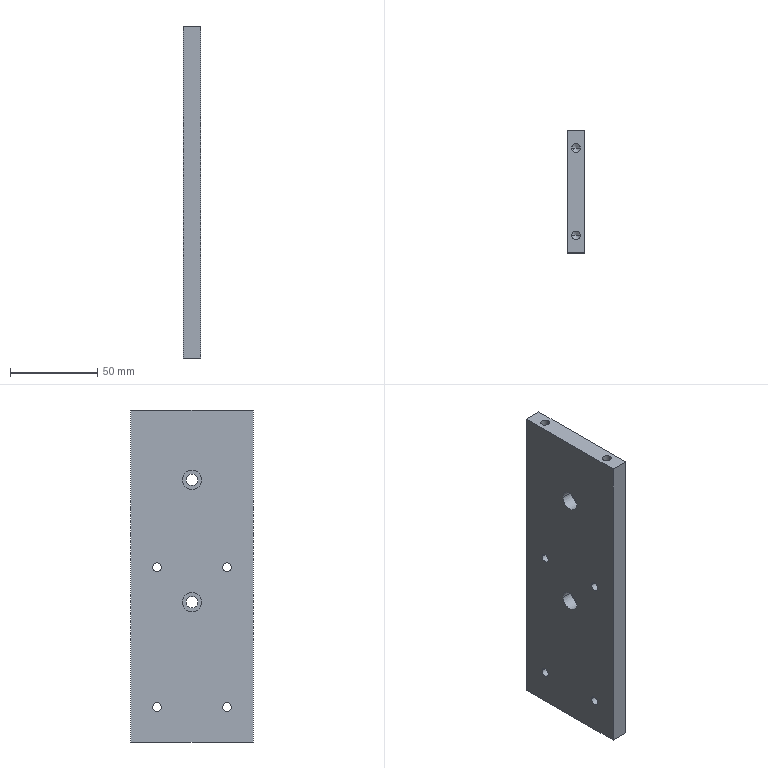Component | SolidWorks | 01-05MarkingMachineMountingVerticalPlate-1 | 1 solid | 32 faces | box 10 x 70 x 190 mm | volume 130094 mm3 | cylinder 20 | plane 8 | cone 4 | commonest cylinder face diameters 5 x12 11 x4 6.6 x4 | material A3 Steel
build123d program:
from build123d import *

# Parameters (mm, degrees)
SKETCH1_W                                          = 70
SKETCH1_H                                          = 190
BOSS_EXTRUDE1_DEPTH                                = 5
M6_TAPPED_HOLE1_D                                  = 5
M6_TAPPED_HOLE1_DEPTH                              = 15
M6_TAPPED_HOLE1_TIP                                = 1.502
HOLE_SIZE_ACCORDING_TO_TYPE_1_OF_HEXAG_D           = 6.6
HOLE_SIZE_ACCORDING_TO_TYPE_1_OF_HEXAG_CBORE_D     = 11
HOLE_SIZE_ACCORDING_TO_TYPE_1_OF_HEXAG_CBORE_DEPTH = 6.8
M6_TAPPED_HOLE2_D                                  = 5


with BuildPart() as part:
    # Sketch1 → Boss-Extrude1 (new, symmetric)
    with BuildSketch(Plane.XY):
        Rectangle(SKETCH1_W, SKETCH1_H)
    extrude(amount=BOSS_EXTRUDE1_DEPTH, both=True)

    # M6 Tapped Hole1
    with Locations(Plane(origin=(-25, -95, 0), x_dir=(0, 0, -1), z_dir=(0, -1, 0))):
        with Locations((0, 0), (0, 50)):
            Hole(M6_TAPPED_HOLE1_D / 2, depth=M6_TAPPED_HOLE1_DEPTH)
            with Locations((0, 0, -(M6_TAPPED_HOLE1_DEPTH + M6_TAPPED_HOLE1_TIP / 2))):  # 118° drill point
                Cone(0, M6_TAPPED_HOLE1_D / 2, M6_TAPPED_HOLE1_TIP, mode=Mode.SUBTRACT)

    # Hole Size _According to_ Type 1 of Hexag (through all)
    with Locations(Plane(origin=(0, 15, 5), x_dir=(1, 0, 0), z_dir=(0, 0, 1))):
        with Locations((0, 0), (0, -70)):
            CounterBoreHole(HOLE_SIZE_ACCORDING_TO_TYPE_1_OF_HEXAG_D / 2, HOLE_SIZE_ACCORDING_TO_TYPE_1_OF_HEXAG_CBORE_D / 2, HOLE_SIZE_ACCORDING_TO_TYPE_1_OF_HEXAG_CBORE_DEPTH)

    # M6 Tapped Hole2 (through all)
    with Locations(Plane(origin=(-20, -5, 5), x_dir=(1, 0, 0), z_dir=(0, 0, 1))):
        with Locations((0, 0), (0, 80), (40, 80), (40, 0)):
            Hole(M6_TAPPED_HOLE2_D / 2)


solid = part.part

# Placed as in the assembly
solid = solid.moved(Location((-51.91, 2.41, -10), (-90, -90, 0)))
STEP:
#1=CARTESIAN_POINT('',(-1.847,-0.7909,-0.1969));
#2=VERTEX_POINT('',#1);
#3=CARTESIAN_POINT('',(-1.847,-0.5941,-0.1969));
#4=VERTEX_POINT('',#3);
#5=CARTESIAN_POINT('',(-1.847,-0.6925,-0.1969));
#6=DIRECTION('',(-1.,0.,0.));
#7=DIRECTION('',(0.,1.,0.));
#8=AXIS2_PLACEMENT_3D('',#5,#6,#7);
#9=CIRCLE('',#8,0.09843);
#10=EDGE_CURVE('',#2,#4,#9,.T.);
#11=ORIENTED_EDGE('',*,*,#10,.F.);
#12=CARTESIAN_POINT('',(-2.241,-0.7909,-0.1969));
#13=VERTEX_POINT('',#12);
#14=CARTESIAN_POINT('',(-2.241,-0.7909,-0.1969));
#15=DIRECTION('',(-1.,0.,0.));
#16=VECTOR('',#15,39.37);
#17=LINE('',#14,#16);
#18=EDGE_CURVE('',#2,#13,#17,.T.);
#19=ORIENTED_EDGE('',*,*,#18,.T.);
#20=CARTESIAN_POINT('',(-2.241,-0.5941,-0.1969));
#21=VERTEX_POINT('',#20);
#22=CARTESIAN_POINT('',(-2.241,-0.6925,-0.1969));
#23=DIRECTION('',(-1.,0.,0.));
#24=DIRECTION('',(0.,1.,0.));
#25=AXIS2_PLACEMENT_3D('',#22,#23,#24);
#26=CIRCLE('',#25,0.09843);
#27=EDGE_CURVE('',#13,#21,#26,.T.);
#28=ORIENTED_EDGE('',*,*,#27,.T.);
#29=CARTESIAN_POINT('',(-2.241,-0.5941,-0.1969));
#30=DIRECTION('',(-1.,0.,0.));
#31=VECTOR('',#30,39.37);
#32=LINE('',#29,#31);
#33=EDGE_CURVE('',#4,#21,#32,.T.);
#34=ORIENTED_EDGE('',*,*,#33,.F.);
#35=EDGE_LOOP('',(#11,#19,#28,#34));
#36=FACE_OUTER_BOUND('',#35,.T.);
#37=CARTESIAN_POINT('',(-2.241,-0.6925,-0.1969));
#38=DIRECTION('',(-1.,0.,0.));
#39=DIRECTION('',(0.,1.,0.));
#40=AXIS2_PLACEMENT_3D('',#37,#38,#39);
#41=CYLINDRICAL_SURFACE('',#40,0.09843);
#42=ADVANCED_FACE('',(#36),#41,.F.);
#43=CARTESIAN_POINT('',(-1.847,-0.7909,-3.346));
#44=VERTEX_POINT('',#43);
#45=CARTESIAN_POINT('',(-1.847,-0.5941,-3.346));
#46=VERTEX_POINT('',#45);
#47=CARTESIAN_POINT('',(-1.847,-0.6925,-3.346));
#48=DIRECTION('',(-1.,0.,0.));
#49=DIRECTION('',(0.,1.,0.));
#50=AXIS2_PLACEMENT_3D('',#47,#48,#49);
#51=CIRCLE('',#50,0.09843);
#52=EDGE_CURVE('',#44,#46,#51,.T.);
#53=ORIENTED_EDGE('',*,*,#52,.F.);
#54=CARTESIAN_POINT('',(-2.241,-0.7909,-3.346));
#55=VERTEX_POINT('',#54);
#56=CARTESIAN_POINT('',(-2.241,-0.7909,-3.346));
#57=DIRECTION('',(-1.,0.,0.));
#58=VECTOR('',#57,39.37);
#59=LINE('',#56,#58);
#60=EDGE_CURVE('',#44,#55,#59,.T.);
#61=ORIENTED_EDGE('',*,*,#60,.T.);
#62=CARTESIAN_POINT('',(-2.241,-0.5941,-3.346));
#63=VERTEX_POINT('',#62);
#64=CARTESIAN_POINT('',(-2.241,-0.6925,-3.346));
#65=DIRECTION('',(-1.,0.,0.));
#66=DIRECTION('',(0.,1.,0.));
#67=AXIS2_PLACEMENT_3D('',#64,#65,#66);
#68=CIRCLE('',#67,0.09843);
#69=EDGE_CURVE('',#55,#63,#68,.T.);
#70=ORIENTED_EDGE('',*,*,#69,.T.);
#71=CARTESIAN_POINT('',(-2.241,-0.5941,-3.346));
#72=DIRECTION('',(-1.,0.,0.));
#73=VECTOR('',#72,39.37);
#74=LINE('',#71,#73);
#75=EDGE_CURVE('',#46,#63,#74,.T.);
#76=ORIENTED_EDGE('',*,*,#75,.F.);
#77=EDGE_LOOP('',(#53,#61,#70,#76));
#78=FACE_OUTER_BOUND('',#77,.T.);
#79=CARTESIAN_POINT('',(-2.241,-0.6925,-3.346));
#80=DIRECTION('',(-1.,0.,0.));
#81=DIRECTION('',(0.,1.,0.));
#82=AXIS2_PLACEMENT_3D('',#79,#80,#81);
#83=CYLINDRICAL_SURFACE('',#82,0.09843);
#84=ADVANCED_FACE('',(#78),#83,.F.);
#85=CARTESIAN_POINT('',(-1.847,0.7839,-3.346));
#86=VERTEX_POINT('',#85);
#87=CARTESIAN_POINT('',(-1.847,0.9807,-3.346));
#88=VERTEX_POINT('',#87);
#89=CARTESIAN_POINT('',(-1.847,0.8823,-3.346));
#90=DIRECTION('',(-1.,0.,0.));
#91=DIRECTION('',(0.,1.,0.));
#92=AXIS2_PLACEMENT_3D('',#89,#90,#91);
#93=CIRCLE('',#92,0.09843);
#94=EDGE_CURVE('',#86,#88,#93,.T.);
#95=ORIENTED_EDGE('',*,*,#94,.F.);
#96=CARTESIAN_POINT('',(-2.241,0.7839,-3.346));
#97=VERTEX_POINT('',#96);
#98=CARTESIAN_POINT('',(-2.241,0.7839,-3.346));
#99=DIRECTION('',(-1.,0.,0.));
#100=VECTOR('',#99,39.37);
#101=LINE('',#98,#100);
#102=EDGE_CURVE('',#86,#97,#101,.T.);
#103=ORIENTED_EDGE('',*,*,#102,.T.);
#104=CARTESIAN_POINT('',(-2.241,0.9807,-3.346));
#105=VERTEX_POINT('',#104);
#106=CARTESIAN_POINT('',(-2.241,0.8823,-3.346));
#107=DIRECTION('',(-1.,0.,0.));
#108=DIRECTION('',(0.,1.,0.));
#109=AXIS2_PLACEMENT_3D('',#106,#107,#108);
#110=CIRCLE('',#109,0.09843);
#111=EDGE_CURVE('',#97,#105,#110,.T.);
#112=ORIENTED_EDGE('',*,*,#111,.T.);
#113=CARTESIAN_POINT('',(-2.241,0.9807,-3.346));
#114=DIRECTION('',(-1.,0.,0.));
#115=VECTOR('',#114,39.37);
#116=LINE('',#113,#115);
#117=EDGE_CURVE('',#88,#105,#116,.T.);
#118=ORIENTED_EDGE('',*,*,#117,.F.);
#119=EDGE_LOOP('',(#95,#103,#112,#118));
#120=FACE_OUTER_BOUND('',#119,.T.);
#121=CARTESIAN_POINT('',(-2.241,0.8823,-3.346));
#122=DIRECTION('',(-1.,0.,0.));
#123=DIRECTION('',(0.,1.,0.));
#124=AXIS2_PLACEMENT_3D('',#121,#122,#123);
#125=CYLINDRICAL_SURFACE('',#124,0.09843);
#126=ADVANCED_FACE('',(#120),#125,.F.);
#127=CARTESIAN_POINT('',(-1.847,0.7839,-0.1969));
#128=VERTEX_POINT('',#127);
#129=CARTESIAN_POINT('',(-1.847,0.9807,-0.1969));
#130=VERTEX_POINT('',#129);
#131=CARTESIAN_POINT('',(-1.847,0.8823,-0.1969));
#132=DIRECTION('',(-1.,0.,0.));
#133=DIRECTION('',(0.,1.,0.));
#134=AXIS2_PLACEMENT_3D('',#131,#132,#133);
#135=CIRCLE('',#134,0.09843);
#136=EDGE_CURVE('',#128,#130,#135,.T.);
#137=ORIENTED_EDGE('',*,*,#136,.F.);
#138=CARTESIAN_POINT('',(-2.241,0.7839,-0.1969));
#139=VERTEX_POINT('',#138);
#140=CARTESIAN_POINT('',(-2.241,0.7839,-0.1969));
#141=DIRECTION('',(-1.,0.,0.));
#142=VECTOR('',#141,39.37);
#143=LINE('',#140,#142);
#144=EDGE_CURVE('',#128,#139,#143,.T.);
#145=ORIENTED_EDGE('',*,*,#144,.T.);
#146=CARTESIAN_POINT('',(-2.241,0.9807,-0.1969));
#147=VERTEX_POINT('',#146);
#148=CARTESIAN_POINT('',(-2.241,0.8823,-0.1969));
#149=DIRECTION('',(-1.,0.,0.));
#150=DIRECTION('',(0.,1.,0.));
#151=AXIS2_PLACEMENT_3D('',#148,#149,#150);
#152=CIRCLE('',#151,0.09843);
#153=EDGE_CURVE('',#139,#147,#152,.T.);
#154=ORIENTED_EDGE('',*,*,#153,.T.);
#155=CARTESIAN_POINT('',(-2.241,0.9807,-0.1969));
#156=DIRECTION('',(-1.,0.,0.));
#157=VECTOR('',#156,39.37);
#158=LINE('',#155,#157);
#159=EDGE_CURVE('',#130,#147,#158,.T.);
#160=ORIENTED_EDGE('',*,*,#159,.F.);
#161=EDGE_LOOP('',(#137,#145,#154,#160));
#162=FACE_OUTER_BOUND('',#161,.T.);
#163=CARTESIAN_POINT('',(-2.241,0.8823,-0.1969));
#164=DIRECTION('',(-1.,0.,0.));
#165=DIRECTION('',(0.,1.,0.));
#166=AXIS2_PLACEMENT_3D('',#163,#164,#165);
#167=CYLINDRICAL_SURFACE('',#166,0.09843);
#168=ADVANCED_FACE('',(#162),#167,.F.);
#169=CARTESIAN_POINT('',(-1.973,-0.1216,-0.9843));
#170=VERTEX_POINT('',#169);
#171=CARTESIAN_POINT('',(-1.973,0.3114,-0.9843));
#172=VERTEX_POINT('',#171);
#173=CARTESIAN_POINT('',(-1.973,0.0949,-0.9843));
#174=DIRECTION('',(-1.,0.,0.));
#175=DIRECTION('',(0.,1.,0.));
#176=AXIS2_PLACEMENT_3D('',#173,#174,#175);
#177=CIRCLE('',#176,0.2165);
#178=EDGE_CURVE('',#170,#172,#177,.T.);
#179=ORIENTED_EDGE('',*,*,#178,.F.);
#180=CARTESIAN_POINT('',(-2.241,-0.1216,-0.9843));
#181=VERTEX_POINT('',#180);
#182=CARTESIAN_POINT('',(-2.241,-0.1216,-0.9843));
#183=DIRECTION('',(-1.,0.,0.));
#184=VECTOR('',#183,39.37);
#185=LINE('',#182,#184);
#186=EDGE_CURVE('',#170,#181,#185,.T.);
#187=ORIENTED_EDGE('',*,*,#186,.T.);
#188=CARTESIAN_POINT('',(-2.241,0.3114,-0.9843));
#189=VERTEX_POINT('',#188);
#190=CARTESIAN_POINT('',(-2.241,0.0949,-0.9843));
#191=DIRECTION('',(-1.,0.,0.));
#192=DIRECTION('',(0.,1.,0.));
#193=AXIS2_PLACEMENT_3D('',#190,#191,#192);
#194=CIRCLE('',#193,0.2165);
#195=EDGE_CURVE('',#181,#189,#194,.T.);
#196=ORIENTED_EDGE('',*,*,#195,.T.);
#197=CARTESIAN_POINT('',(-2.241,0.3114,-0.9843));
#198=DIRECTION('',(-1.,0.,0.));
#199=VECTOR('',#198,39.37);
#200=LINE('',#197,#199);
#201=EDGE_CURVE('',#172,#189,#200,.T.);
#202=ORIENTED_EDGE('',*,*,#201,.F.);
#203=EDGE_LOOP('',(#179,#187,#196,#202));
#204=FACE_OUTER_BOUND('',#203,.T.);
#205=CARTESIAN_POINT('',(-2.241,0.0949,-0.9843));
#206=DIRECTION('',(-1.,0.,0.));
#207=DIRECTION('',(0.,1.,0.));
#208=AXIS2_PLACEMENT_3D('',#205,#206,#207);
#209=CYLINDRICAL_SURFACE('',#208,0.2165);
#210=ADVANCED_FACE('',(#204),#209,.F.);
#211=CARTESIAN_POINT('',(-1.847,-0.03502,-0.9843));
#212=VERTEX_POINT('',#211);
#213=CARTESIAN_POINT('',(-1.847,0.2248,-0.9843));
#214=VERTEX_POINT('',#213);
#215=CARTESIAN_POINT('',(-1.847,0.0949,-0.9843));
#216=DIRECTION('',(-1.,0.,0.));
#217=DIRECTION('',(0.,1.,0.));
#218=AXIS2_PLACEMENT_3D('',#215,#216,#217);
#219=CIRCLE('',#218,0.1299);
#220=EDGE_CURVE('',#212,#214,#219,.T.);
#221=ORIENTED_EDGE('',*,*,#220,.F.);
#222=CARTESIAN_POINT('',(-1.973,-0.03502,-0.9843));
#223=VERTEX_POINT('',#222);
#224=CARTESIAN_POINT('',(-2.241,-0.03502,-0.9843));
#225=DIRECTION('',(-1.,0.,0.));
#226=VECTOR('',#225,39.37);
#227=LINE('',#224,#226);
#228=EDGE_CURVE('',#212,#223,#227,.T.);
#229=ORIENTED_EDGE('',*,*,#228,.T.);
#230=CARTESIAN_POINT('',(-1.973,0.2248,-0.9843));
#231=VERTEX_POINT('',#230);
#232=CARTESIAN_POINT('',(-1.973,0.0949,-0.9843));
#233=DIRECTION('',(-1.,0.,0.));
#234=DIRECTION('',(0.,1.,0.));
#235=AXIS2_PLACEMENT_3D('',#232,#233,#234);
#236=CIRCLE('',#235,0.1299);
#237=EDGE_CURVE('',#223,#231,#236,.T.);
#238=ORIENTED_EDGE('',*,*,#237,.T.);
#239=CARTESIAN_POINT('',(-2.241,0.2248,-0.9843));
#240=DIRECTION('',(-1.,0.,0.));
#241=VECTOR('',#240,39.37);
#242=LINE('',#239,#241);
#243=EDGE_CURVE('',#214,#231,#242,.T.);
#244=ORIENTED_EDGE('',*,*,#243,.F.);
#245=EDGE_LOOP('',(#221,#229,#238,#244));
#246=FACE_OUTER_BOUND('',#245,.T.);
#247=CARTESIAN_POINT('',(-2.241,0.0949,-0.9843));
#248=DIRECTION('',(-1.,0.,0.));
#249=DIRECTION('',(0.,1.,0.));
#250=AXIS2_PLACEMENT_3D('',#247,#248,#249);
#251=CYLINDRICAL_SURFACE('',#250,0.1299);
#252=ADVANCED_FACE('',(#246),#251,.F.);
#253=CARTESIAN_POINT('',(-1.973,-0.1216,1.772));
#254=VERTEX_POINT('',#253);
#255=CARTESIAN_POINT('',(-1.973,0.3114,1.772));
#256=VERTEX_POINT('',#255);
#257=CARTESIAN_POINT('',(-1.973,0.0949,1.772));
#258=DIRECTION('',(-1.,0.,0.));
#259=DIRECTION('',(0.,1.,0.));
#260=AXIS2_PLACEMENT_3D('',#257,#258,#259);
#261=CIRCLE('',#260,0.2165);
#262=EDGE_CURVE('',#254,#256,#261,.T.);
#263=ORIENTED_EDGE('',*,*,#262,.F.);
#264=CARTESIAN_POINT('',(-2.241,-0.1216,1.772));
#265=VERTEX_POINT('',#264);
#266=CARTESIAN_POINT('',(-2.241,-0.1216,1.772));
#267=DIRECTION('',(-1.,0.,0.));
#268=VECTOR('',#267,39.37);
#269=LINE('',#266,#268);
#270=EDGE_CURVE('',#254,#265,#269,.T.);
#271=ORIENTED_EDGE('',*,*,#270,.T.);
#272=CARTESIAN_POINT('',(-2.241,0.3114,1.772));
#273=VERTEX_POINT('',#272);
#274=CARTESIAN_POINT('',(-2.241,0.0949,1.772));
#275=DIRECTION('',(-1.,0.,0.));
#276=DIRECTION('',(0.,1.,0.));
#277=AXIS2_PLACEMENT_3D('',#274,#275,#276);
#278=CIRCLE('',#277,0.2165);
#279=EDGE_CURVE('',#265,#273,#278,.T.);
#280=ORIENTED_EDGE('',*,*,#279,.T.);
#281=CARTESIAN_POINT('',(-2.241,0.3114,1.772));
#282=DIRECTION('',(-1.,0.,0.));
#283=VECTOR('',#282,39.37);
#284=LINE('',#281,#283);
#285=EDGE_CURVE('',#256,#273,#284,.T.);
#286=ORIENTED_EDGE('',*,*,#285,.F.);
#287=EDGE_LOOP('',(#263,#271,#280,#286));
#288=FACE_OUTER_BOUND('',#287,.T.);
#289=CARTESIAN_POINT('',(-2.241,0.0949,1.772));
#290=DIRECTION('',(-1.,0.,0.));
#291=DIRECTION('',(0.,1.,0.));
#292=AXIS2_PLACEMENT_3D('',#289,#290,#291);
#293=CYLINDRICAL_SURFACE('',#292,0.2165);
#294=ADVANCED_FACE('',(#288),#293,.F.);
#295=CARTESIAN_POINT('',(-1.847,-0.03502,1.772));
#296=VERTEX_POINT('',#295);
#297=CARTESIAN_POINT('',(-1.847,0.2248,1.772));
#298=VERTEX_POINT('',#297);
#299=CARTESIAN_POINT('',(-1.847,0.0949,1.772));
#300=DIRECTION('',(-1.,0.,0.));
#301=DIRECTION('',(0.,1.,0.));
#302=AXIS2_PLACEMENT_3D('',#299,#300,#301);
#303=CIRCLE('',#302,0.1299);
#304=EDGE_CURVE('',#296,#298,#303,.T.);
#305=ORIENTED_EDGE('',*,*,#304,.F.);
#306=CARTESIAN_POINT('',(-1.973,-0.03502,1.772));
#307=VERTEX_POINT('',#306);
#308=CARTESIAN_POINT('',(-2.241,-0.03502,1.772));
#309=DIRECTION('',(-1.,0.,0.));
#310=VECTOR('',#309,39.37);
#311=LINE('',#308,#310);
#312=EDGE_CURVE('',#296,#307,#311,.T.);
#313=ORIENTED_EDGE('',*,*,#312,.T.);
#314=CARTESIAN_POINT('',(-1.973,0.2248,1.772));
#315=VERTEX_POINT('',#314);
#316=CARTESIAN_POINT('',(-1.973,0.0949,1.772));
#317=DIRECTION('',(-1.,0.,0.));
#318=DIRECTION('',(0.,1.,0.));
#319=AXIS2_PLACEMENT_3D('',#316,#317,#318);
#320=CIRCLE('',#319,0.1299);
#321=EDGE_CURVE('',#307,#315,#320,.T.);
#322=ORIENTED_EDGE('',*,*,#321,.T.);
#323=CARTESIAN_POINT('',(-2.241,0.2248,1.772));
#324=DIRECTION('',(-1.,0.,0.));
#325=VECTOR('',#324,39.37);
#326=LINE('',#323,#325);
#327=EDGE_CURVE('',#298,#315,#326,.T.);
#328=ORIENTED_EDGE('',*,*,#327,.F.);
#329=EDGE_LOOP('',(#305,#313,#322,#328));
#330=FACE_OUTER_BOUND('',#329,.T.);
#331=CARTESIAN_POINT('',(-2.241,0.0949,1.772));
#332=DIRECTION('',(-1.,0.,0.));
#333=DIRECTION('',(0.,1.,0.));
#334=AXIS2_PLACEMENT_3D('',#331,#332,#333);
#335=CYLINDRICAL_SURFACE('',#334,0.1299);
#336=ADVANCED_FACE('',(#330),#335,.F.);
#337=CARTESIAN_POINT('',(-2.142,-0.8894,2.756));
#338=VERTEX_POINT('',#337);
#339=CARTESIAN_POINT('',(-1.945,-0.8894,2.756));
#340=VERTEX_POINT('',#339);
#341=CARTESIAN_POINT('',(-2.044,-0.8894,2.756));
#342=DIRECTION('',(0.,-0.,1.));
#343=DIRECTION('',(1.,0.,0.));
#344=AXIS2_PLACEMENT_3D('',#341,#342,#343);
#345=CIRCLE('',#344,0.09843);
#346=EDGE_CURVE('',#338,#340,#345,.T.);
#347=ORIENTED_EDGE('',*,*,#346,.F.);
#348=CARTESIAN_POINT('',(-2.142,-0.8894,3.346));
#349=VERTEX_POINT('',#348);
#350=CARTESIAN_POINT('',(-2.142,-0.8894,3.346));
#351=DIRECTION('',(0.,-0.,1.));
#352=VECTOR('',#351,39.37);
#353=LINE('',#350,#352);
#354=EDGE_CURVE('',#338,#349,#353,.T.);
#355=ORIENTED_EDGE('',*,*,#354,.T.);
#356=CARTESIAN_POINT('',(-1.945,-0.8894,3.346));
#357=VERTEX_POINT('',#356);
#358=CARTESIAN_POINT('',(-2.044,-0.8894,3.346));
#359=DIRECTION('',(0.,-0.,1.));
#360=DIRECTION('',(1.,0.,0.));
#361=AXIS2_PLACEMENT_3D('',#358,#359,#360);
#362=CIRCLE('',#361,0.09843);
#363=EDGE_CURVE('',#349,#357,#362,.T.);
#364=ORIENTED_EDGE('',*,*,#363,.T.);
#365=CARTESIAN_POINT('',(-1.945,-0.8894,3.346));
#366=DIRECTION('',(0.,-0.,1.));
#367=VECTOR('',#366,39.37);
#368=LINE('',#365,#367);
#369=EDGE_CURVE('',#340,#357,#368,.T.);
#370=ORIENTED_EDGE('',*,*,#369,.F.);
#371=EDGE_LOOP('',(#347,#355,#364,#370));
#372=FACE_OUTER_BOUND('',#371,.T.);
#373=CARTESIAN_POINT('',(-2.044,-0.8894,3.346));
#374=DIRECTION('',(0.,-0.,1.));
#375=DIRECTION('',(1.,0.,0.));
#376=AXIS2_PLACEMENT_3D('',#373,#374,#375);
#377=CYLINDRICAL_SURFACE('',#376,0.09843);
#378=ADVANCED_FACE('',(#372),#377,.F.);
#379=CARTESIAN_POINT('',(-2.044,-0.8894,2.697));
#380=VERTEX_POINT('',#379);
#381=CARTESIAN_POINT('',(-1.945,-0.8894,2.756));
#382=DIRECTION('',(0.8572,-0.,0.515));
#383=VECTOR('',#382,39.37);
#384=LINE('',#381,#383);
#385=EDGE_CURVE('',#380,#340,#384,.T.);
#386=ORIENTED_EDGE('',*,*,#385,.F.);
#387=CARTESIAN_POINT('',(-2.142,-0.8894,2.756));
#388=DIRECTION('',(-0.8572,0.,0.515));
#389=VECTOR('',#388,39.37);
#390=LINE('',#387,#389);
#391=EDGE_CURVE('',#380,#338,#390,.T.);
#392=ORIENTED_EDGE('',*,*,#391,.T.);
#393=ORIENTED_EDGE('',*,*,#346,.T.);
#394=EDGE_LOOP('',(#386,#392,#393));
#395=FACE_OUTER_BOUND('',#394,.T.);
#396=CARTESIAN_POINT('',(-2.044,-0.8894,2.756));
#397=DIRECTION('',(0.,-0.,1.));
#398=DIRECTION('',(1.,0.,0.));
#399=AXIS2_PLACEMENT_3D('',#396,#397,#398);
#400=CONICAL_SURFACE('',#399,0.09843,1.03);
#401=ADVANCED_FACE('',(#395),#400,.F.);
#402=CARTESIAN_POINT('',(-2.142,1.079,2.756));
#403=VERTEX_POINT('',#402);
#404=CARTESIAN_POINT('',(-1.945,1.079,2.756));
#405=VERTEX_POINT('',#404);
#406=CARTESIAN_POINT('',(-2.044,1.079,2.756));
#407=DIRECTION('',(0.,-0.,1.));
#408=DIRECTION('',(1.,0.,0.));
#409=AXIS2_PLACEMENT_3D('',#406,#407,#408);
#410=CIRCLE('',#409,0.09843);
#411=EDGE_CURVE('',#403,#405,#410,.T.);
#412=ORIENTED_EDGE('',*,*,#411,.F.);
#413=CARTESIAN_POINT('',(-2.142,1.079,3.346));
#414=VERTEX_POINT('',#413);
#415=CARTESIAN_POINT('',(-2.142,1.079,3.346));
#416=DIRECTION('',(0.,-0.,1.));
#417=VECTOR('',#416,39.37);
#418=LINE('',#415,#417);
#419=EDGE_CURVE('',#403,#414,#418,.T.);
#420=ORIENTED_EDGE('',*,*,#419,.T.);
#421=CARTESIAN_POINT('',(-1.945,1.079,3.346));
#422=VERTEX_POINT('',#421);
#423=CARTESIAN_POINT('',(-2.044,1.079,3.346));
#424=DIRECTION('',(0.,-0.,1.));
#425=DIRECTION('',(1.,0.,0.));
#426=AXIS2_PLACEMENT_3D('',#423,#424,#425);
#427=CIRCLE('',#426,0.09843);
#428=EDGE_CURVE('',#414,#422,#427,.T.);
#429=ORIENTED_EDGE('',*,*,#428,.T.);
#430=CARTESIAN_POINT('',(-1.945,1.079,3.346));
#431=DIRECTION('',(0.,-0.,1.));
#432=VECTOR('',#431,39.37);
#433=LINE('',#430,#432);
#434=EDGE_CURVE('',#405,#422,#433,.T.);
#435=ORIENTED_EDGE('',*,*,#434,.F.);
#436=EDGE_LOOP('',(#412,#420,#429,#435));
#437=FACE_OUTER_BOUND('',#436,.T.);
#438=CARTESIAN_POINT('',(-2.044,1.079,3.346));
#439=DIRECTION('',(0.,-0.,1.));
#440=DIRECTION('',(1.,0.,0.));
#441=AXIS2_PLACEMENT_3D('',#438,#439,#440);
#442=CYLINDRICAL_SURFACE('',#441,0.09843);
#443=ADVANCED_FACE('',(#437),#442,.F.);
#444=CARTESIAN_POINT('',(-2.044,1.079,2.697));
#445=VERTEX_POINT('',#444);
#446=CARTESIAN_POINT('',(-1.945,1.079,2.756));
#447=DIRECTION('',(0.8572,-0.,0.515));
#448=VECTOR('',#447,39.37);
#449=LINE('',#446,#448);
#450=EDGE_CURVE('',#445,#405,#449,.T.);
#451=ORIENTED_EDGE('',*,*,#450,.F.);
#452=CARTESIAN_POINT('',(-2.142,1.079,2.756));
#453=DIRECTION('',(-0.8572,0.,0.515));
#454=VECTOR('',#453,39.37);
#455=LINE('',#452,#454);
#456=EDGE_CURVE('',#445,#403,#455,.T.);
#457=ORIENTED_EDGE('',*,*,#456,.T.);
#458=ORIENTED_EDGE('',*,*,#411,.T.);
#459=EDGE_LOOP('',(#451,#457,#458));
#460=FACE_OUTER_BOUND('',#459,.T.);
#461=CARTESIAN_POINT('',(-2.044,1.079,2.756));
#462=DIRECTION('',(0.,-0.,1.));
#463=DIRECTION('',(1.,0.,0.));
#464=AXIS2_PLACEMENT_3D('',#461,#462,#463);
#465=CONICAL_SURFACE('',#464,0.09843,1.03);
#466=ADVANCED_FACE('',(#460),#465,.F.);
#467=CARTESIAN_POINT('',(-2.241,-0.6925,-0.1969));
#468=DIRECTION('',(-1.,0.,0.));
#469=DIRECTION('',(0.,1.,0.));
#470=AXIS2_PLACEMENT_3D('',#467,#468,#469);
#471=CIRCLE('',#470,0.09843);
#472=EDGE_CURVE('',#21,#13,#471,.T.);
#473=ORIENTED_EDGE('',*,*,#472,.F.);
#474=ORIENTED_EDGE('',*,*,#27,.F.);
#475=EDGE_LOOP('',(#473,#474));
#476=FACE_BOUND('',#475,.T.);
#477=CARTESIAN_POINT('',(-2.241,-0.6925,-3.346));
#478=DIRECTION('',(-1.,0.,0.));
#479=DIRECTION('',(0.,1.,0.));
#480=AXIS2_PLACEMENT_3D('',#477,#478,#479);
#481=CIRCLE('',#480,0.09843);
#482=EDGE_CURVE('',#63,#55,#481,.T.);
#483=ORIENTED_EDGE('',*,*,#482,.F.);
#484=ORIENTED_EDGE('',*,*,#69,.F.);
#485=EDGE_LOOP('',(#483,#484));
#486=FACE_BOUND('',#485,.T.);
#487=CARTESIAN_POINT('',(-2.241,0.8823,-3.346));
#488=DIRECTION('',(-1.,0.,0.));
#489=DIRECTION('',(0.,1.,0.));
#490=AXIS2_PLACEMENT_3D('',#487,#488,#489);
#491=CIRCLE('',#490,0.09843);
#492=EDGE_CURVE('',#105,#97,#491,.T.);
#493=ORIENTED_EDGE('',*,*,#492,.F.);
#494=ORIENTED_EDGE('',*,*,#111,.F.);
#495=EDGE_LOOP('',(#493,#494));
#496=FACE_BOUND('',#495,.T.);
#497=CARTESIAN_POINT('',(-2.241,0.8823,-0.1969));
#498=DIRECTION('',(-1.,0.,0.));
#499=DIRECTION('',(0.,1.,0.));
#500=AXIS2_PLACEMENT_3D('',#497,#498,#499);
#501=CIRCLE('',#500,0.09843);
#502=EDGE_CURVE('',#147,#139,#501,.T.);
#503=ORIENTED_EDGE('',*,*,#502,.F.);
#504=ORIENTED_EDGE('',*,*,#153,.F.);
#505=EDGE_LOOP('',(#503,#504));
#506=FACE_BOUND('',#505,.T.);
#507=CARTESIAN_POINT('',(-2.241,0.0949,1.772));
#508=DIRECTION('',(-1.,0.,0.));
#509=DIRECTION('',(0.,1.,0.));
#510=AXIS2_PLACEMENT_3D('',#507,#508,#509);
#511=CIRCLE('',#510,0.2165);
#512=EDGE_CURVE('',#273,#265,#511,.T.);
#513=ORIENTED_EDGE('',*,*,#512,.F.);
#514=ORIENTED_EDGE('',*,*,#279,.F.);
#515=EDGE_LOOP('',(#513,#514));
#516=FACE_BOUND('',#515,.T.);
#517=CARTESIAN_POINT('',(-2.241,1.473,3.346));
#518=VERTEX_POINT('',#517);
#519=CARTESIAN_POINT('',(-2.241,1.473,-4.134));
#520=VERTEX_POINT('',#519);
#521=CARTESIAN_POINT('',(-2.241,1.473,3.346));
#522=DIRECTION('',(-0.,0.,-1.));
#523=VECTOR('',#522,39.37);
#524=LINE('',#521,#523);
#525=EDGE_CURVE('',#518,#520,#524,.T.);
#526=ORIENTED_EDGE('',*,*,#525,.T.);
#527=CARTESIAN_POINT('',(-2.241,-1.283,-4.134));
#528=VERTEX_POINT('',#527);
#529=CARTESIAN_POINT('',(-2.241,-1.283,-4.134));
#530=DIRECTION('',(-0.,-1.,0.));
#531=VECTOR('',#530,39.37);
#532=LINE('',#529,#531);
#533=EDGE_CURVE('',#520,#528,#532,.T.);
#534=ORIENTED_EDGE('',*,*,#533,.T.);
#535=CARTESIAN_POINT('',(-2.241,-1.283,3.346));
#536=VERTEX_POINT('',#535);
#537=CARTESIAN_POINT('',(-2.241,-1.283,3.346));
#538=DIRECTION('',(0.,-0.,1.));
#539=VECTOR('',#538,39.37);
#540=LINE('',#537,#539);
#541=EDGE_CURVE('',#528,#536,#540,.T.);
#542=ORIENTED_EDGE('',*,*,#541,.T.);
#543=CARTESIAN_POINT('',(-2.241,-1.283,3.346));
#544=DIRECTION('',(0.,1.,0.));
#545=VECTOR('',#544,39.37);
#546=LINE('',#543,#545);
#547=EDGE_CURVE('',#536,#518,#546,.T.);
#548=ORIENTED_EDGE('',*,*,#547,.T.);
#549=EDGE_LOOP('',(#526,#534,#542,#548));
#550=FACE_OUTER_BOUND('',#549,.T.);
#551=CARTESIAN_POINT('',(-2.241,0.0949,-0.9843));
#552=DIRECTION('',(-1.,0.,0.));
#553=DIRECTION('',(0.,1.,0.));
#554=AXIS2_PLACEMENT_3D('',#551,#552,#553);
#555=CIRCLE('',#554,0.2165);
#556=EDGE_CURVE('',#189,#181,#555,.T.);
#557=ORIENTED_EDGE('',*,*,#556,.F.);
#558=ORIENTED_EDGE('',*,*,#195,.F.);
#559=EDGE_LOOP('',(#557,#558));
#560=FACE_BOUND('',#559,.T.);
#561=CARTESIAN_POINT('',(-2.241,0.0949,-0.3937));
#562=DIRECTION('',(1.,-0.,-0.));
#563=DIRECTION('',(-0.,-1.,0.));
#564=AXIS2_PLACEMENT_3D('',#561,#562,#563);
#565=PLANE('',#564);
#566=ADVANCED_FACE('',(#476,#486,#496,#506,#516,#550,#560),#565,.F.);
#567=CARTESIAN_POINT('',(-1.847,1.473,3.346));
#568=VERTEX_POINT('',#567);
#569=CARTESIAN_POINT('',(-1.847,1.473,-4.134));
#570=VERTEX_POINT('',#569);
#571=CARTESIAN_POINT('',(-1.847,1.473,3.346));
#572=DIRECTION('',(-0.,0.,-1.));
#573=VECTOR('',#572,39.37);
#574=LINE('',#571,#573);
#575=EDGE_CURVE('',#568,#570,#574,.T.);
#576=ORIENTED_EDGE('',*,*,#575,.T.);
#577=CARTESIAN_POINT('',(-2.241,1.473,-4.134));
#578=DIRECTION('',(1.,-0.,-0.));
#579=VECTOR('',#578,39.37);
#580=LINE('',#577,#579);
#581=EDGE_CURVE('',#520,#570,#580,.T.);
#582=ORIENTED_EDGE('',*,*,#581,.F.);
#583=ORIENTED_EDGE('',*,*,#525,.F.);
#584=CARTESIAN_POINT('',(-2.241,1.473,3.346));
#585=DIRECTION('',(1.,-0.,-0.));
#586=VECTOR('',#585,39.37);
#587=LINE('',#584,#586);
#588=EDGE_CURVE('',#518,#568,#587,.T.);
#589=ORIENTED_EDGE('',*,*,#588,.T.);
#590=EDGE_LOOP('',(#576,#582,#583,#589));
#591=FACE_OUTER_BOUND('',#590,.T.);
#592=CARTESIAN_POINT('',(-2.241,1.473,3.346));
#593=DIRECTION('',(-0.,-1.,0.));
#594=DIRECTION('',(-1.,0.,0.));
#595=AXIS2_PLACEMENT_3D('',#592,#593,#594);
#596=PLANE('',#595);
#597=ADVANCED_FACE('',(#591),#596,.F.);
#598=CARTESIAN_POINT('',(-1.847,-1.283,-4.134));
#599=VERTEX_POINT('',#598);
#600=CARTESIAN_POINT('',(-1.847,-1.283,-4.134));
#601=DIRECTION('',(-0.,-1.,0.));
#602=VECTOR('',#601,39.37);
#603=LINE('',#600,#602);
#604=EDGE_CURVE('',#570,#599,#603,.T.);
#605=ORIENTED_EDGE('',*,*,#604,.T.);
#606=CARTESIAN_POINT('',(-2.241,-1.283,-4.134));
#607=DIRECTION('',(1.,-0.,-0.));
#608=VECTOR('',#607,39.37);
#609=LINE('',#606,#608);
#610=EDGE_CURVE('',#528,#599,#609,.T.);
#611=ORIENTED_EDGE('',*,*,#610,.F.);
#612=ORIENTED_EDGE('',*,*,#533,.F.);
#613=ORIENTED_EDGE('',*,*,#581,.T.);
#614=EDGE_LOOP('',(#605,#611,#612,#613));
#615=FACE_OUTER_BOUND('',#614,.T.);
#616=CARTESIAN_POINT('',(-2.241,-1.283,-4.134));
#617=DIRECTION('',(0.,-0.,1.));
#618=DIRECTION('',(1.,-0.,-0.));
#619=AXIS2_PLACEMENT_3D('',#616,#617,#618);
#620=PLANE('',#619);
#621=ADVANCED_FACE('',(#615),#620,.F.);
#622=CARTESIAN_POINT('',(-1.847,-1.283,3.346));
#623=VERTEX_POINT('',#622);
#624=CARTESIAN_POINT('',(-1.847,-1.283,3.346));
#625=DIRECTION('',(0.,-0.,1.));
#626=VECTOR('',#625,39.37);
#627=LINE('',#624,#626);
#628=EDGE_CURVE('',#599,#623,#627,.T.);
#629=ORIENTED_EDGE('',*,*,#628,.T.);
#630=CARTESIAN_POINT('',(-2.241,-1.283,3.346));
#631=DIRECTION('',(1.,-0.,-0.));
#632=VECTOR('',#631,39.37);
#633=LINE('',#630,#632);
#634=EDGE_CURVE('',#536,#623,#633,.T.);
#635=ORIENTED_EDGE('',*,*,#634,.F.);
#636=ORIENTED_EDGE('',*,*,#541,.F.);
#637=ORIENTED_EDGE('',*,*,#610,.T.);
#638=EDGE_LOOP('',(#629,#635,#636,#637));
#639=FACE_OUTER_BOUND('',#638,.T.);
#640=CARTESIAN_POINT('',(-2.241,-1.283,3.346));
#641=DIRECTION('',(0.,1.,0.));
#642=DIRECTION('',(1.,-0.,-0.));
#643=AXIS2_PLACEMENT_3D('',#640,#641,#642);
#644=PLANE('',#643);
#645=ADVANCED_FACE('',(#639),#644,.F.);
#646=CARTESIAN_POINT('',(-2.044,-0.8894,3.346));
#647=DIRECTION('',(0.,-0.,1.));
#648=DIRECTION('',(1.,0.,0.));
#649=AXIS2_PLACEMENT_3D('',#646,#647,#648);
#650=CIRCLE('',#649,0.09843);
#651=EDGE_CURVE('',#357,#349,#650,.T.);
#652=ORIENTED_EDGE('',*,*,#651,.F.);
#653=ORIENTED_EDGE('',*,*,#363,.F.);
#654=EDGE_LOOP('',(#652,#653));
#655=FACE_BOUND('',#654,.T.);
#656=CARTESIAN_POINT('',(-2.044,1.079,3.346));
#657=DIRECTION('',(0.,-0.,1.));
#658=DIRECTION('',(1.,0.,0.));
#659=AXIS2_PLACEMENT_3D('',#656,#657,#658);
#660=CIRCLE('',#659,0.09843);
#661=EDGE_CURVE('',#422,#414,#660,.T.);
#662=ORIENTED_EDGE('',*,*,#661,.F.);
#663=ORIENTED_EDGE('',*,*,#428,.F.);
#664=EDGE_LOOP('',(#662,#663));
#665=FACE_BOUND('',#664,.T.);
#666=CARTESIAN_POINT('',(-1.847,-1.283,3.346));
#667=DIRECTION('',(0.,1.,0.));
#668=VECTOR('',#667,39.37);
#669=LINE('',#666,#668);
#670=EDGE_CURVE('',#623,#568,#669,.T.);
#671=ORIENTED_EDGE('',*,*,#670,.T.);
#672=ORIENTED_EDGE('',*,*,#588,.F.);
#673=ORIENTED_EDGE('',*,*,#547,.F.);
#674=ORIENTED_EDGE('',*,*,#634,.T.);
#675=EDGE_LOOP('',(#671,#672,#673,#674));
#676=FACE_OUTER_BOUND('',#675,.T.);
#677=CARTESIAN_POINT('',(-2.241,-1.283,3.346));
#678=DIRECTION('',(-0.,0.,-1.));
#679=DIRECTION('',(-1.,0.,0.));
#680=AXIS2_PLACEMENT_3D('',#677,#678,#679);
#681=PLANE('',#680);
#682=ADVANCED_FACE('',(#655,#665,#676),#681,.F.);
#683=CARTESIAN_POINT('',(-1.847,-0.6925,-0.1969));
#684=DIRECTION('',(-1.,0.,0.));
#685=DIRECTION('',(0.,1.,0.));
#686=AXIS2_PLACEMENT_3D('',#683,#684,#685);
#687=CIRCLE('',#686,0.09843);
#688=EDGE_CURVE('',#4,#2,#687,.T.);
#689=ORIENTED_EDGE('',*,*,#688,.T.);
#690=ORIENTED_EDGE('',*,*,#10,.T.);
#691=EDGE_LOOP('',(#689,#690));
#692=FACE_BOUND('',#691,.T.);
#693=CARTESIAN_POINT('',(-1.847,-0.6925,-3.346));
#694=DIRECTION('',(-1.,0.,0.));
#695=DIRECTION('',(0.,1.,0.));
#696=AXIS2_PLACEMENT_3D('',#693,#694,#695);
#697=CIRCLE('',#696,0.09843);
#698=EDGE_CURVE('',#46,#44,#697,.T.);
#699=ORIENTED_EDGE('',*,*,#698,.T.);
#700=ORIENTED_EDGE('',*,*,#52,.T.);
#701=EDGE_LOOP('',(#699,#700));
#702=FACE_BOUND('',#701,.T.);
#703=CARTESIAN_POINT('',(-1.847,0.8823,-3.346));
#704=DIRECTION('',(-1.,0.,0.));
#705=DIRECTION('',(0.,1.,0.));
#706=AXIS2_PLACEMENT_3D('',#703,#704,#705);
#707=CIRCLE('',#706,0.09843);
#708=EDGE_CURVE('',#88,#86,#707,.T.);
#709=ORIENTED_EDGE('',*,*,#708,.T.);
#710=ORIENTED_EDGE('',*,*,#94,.T.);
#711=EDGE_LOOP('',(#709,#710));
#712=FACE_BOUND('',#711,.T.);
#713=CARTESIAN_POINT('',(-1.847,0.8823,-0.1969));
#714=DIRECTION('',(-1.,0.,0.));
#715=DIRECTION('',(0.,1.,0.));
#716=AXIS2_PLACEMENT_3D('',#713,#714,#715);
#717=CIRCLE('',#716,0.09843);
#718=EDGE_CURVE('',#130,#128,#717,.T.);
#719=ORIENTED_EDGE('',*,*,#718,.T.);
#720=ORIENTED_EDGE('',*,*,#136,.T.);
#721=EDGE_LOOP('',(#719,#720));
#722=FACE_BOUND('',#721,.T.);
#723=CARTESIAN_POINT('',(-1.847,0.0949,-0.9843));
#724=DIRECTION('',(-1.,0.,0.));
#725=DIRECTION('',(0.,1.,0.));
#726=AXIS2_PLACEMENT_3D('',#723,#724,#725);
#727=CIRCLE('',#726,0.1299);
#728=EDGE_CURVE('',#214,#212,#727,.T.);
#729=ORIENTED_EDGE('',*,*,#728,.T.);
#730=ORIENTED_EDGE('',*,*,#220,.T.);
#731=EDGE_LOOP('',(#729,#730));
#732=FACE_BOUND('',#731,.T.);
#733=CARTESIAN_POINT('',(-1.847,0.0949,1.772));
#734=DIRECTION('',(-1.,0.,0.));
#735=DIRECTION('',(0.,1.,0.));
#736=AXIS2_PLACEMENT_3D('',#733,#734,#735);
#737=CIRCLE('',#736,0.1299);
#738=EDGE_CURVE('',#298,#296,#737,.T.);
#739=ORIENTED_EDGE('',*,*,#738,.T.);
#740=ORIENTED_EDGE('',*,*,#304,.T.);
#741=EDGE_LOOP('',(#739,#740));
#742=FACE_BOUND('',#741,.T.);
#743=ORIENTED_EDGE('',*,*,#575,.F.);
#744=ORIENTED_EDGE('',*,*,#670,.F.);
#745=ORIENTED_EDGE('',*,*,#628,.F.);
#746=ORIENTED_EDGE('',*,*,#604,.F.);
#747=EDGE_LOOP('',(#743,#744,#745,#746));
#748=FACE_OUTER_BOUND('',#747,.T.);
#749=CARTESIAN_POINT('',(-1.847,0.0949,-0.3937));
#750=DIRECTION('',(1.,-0.,-0.));
#751=DIRECTION('',(-0.,-1.,0.));
#752=AXIS2_PLACEMENT_3D('',#749,#750,#751);
#753=PLANE('',#752);
#754=ADVANCED_FACE('',(#692,#702,#712,#722,#732,#742,#748),#753,.T.);
#755=ORIENTED_EDGE('',*,*,#456,.F.);
#756=ORIENTED_EDGE('',*,*,#450,.T.);
#757=CARTESIAN_POINT('',(-2.044,1.079,2.756));
#758=DIRECTION('',(0.,-0.,1.));
#759=DIRECTION('',(1.,0.,0.));
#760=AXIS2_PLACEMENT_3D('',#757,#758,#759);
#761=CIRCLE('',#760,0.09843);
#762=EDGE_CURVE('',#405,#403,#761,.T.);
#763=ORIENTED_EDGE('',*,*,#762,.T.);
#764=EDGE_LOOP('',(#755,#756,#763));
#765=FACE_OUTER_BOUND('',#764,.T.);
#766=CARTESIAN_POINT('',(-2.044,1.079,2.756));
#767=DIRECTION('',(0.,-0.,1.));
#768=DIRECTION('',(1.,0.,0.));
#769=AXIS2_PLACEMENT_3D('',#766,#767,#768);
#770=CONICAL_SURFACE('',#769,0.09843,1.03);
#771=ADVANCED_FACE('',(#765),#770,.F.);
#772=ORIENTED_EDGE('',*,*,#419,.F.);
#773=ORIENTED_EDGE('',*,*,#762,.F.);
#774=ORIENTED_EDGE('',*,*,#434,.T.);
#775=ORIENTED_EDGE('',*,*,#661,.T.);
#776=EDGE_LOOP('',(#772,#773,#774,#775));
#777=FACE_OUTER_BOUND('',#776,.T.);
#778=CARTESIAN_POINT('',(-2.044,1.079,3.346));
#779=DIRECTION('',(0.,-0.,1.));
#780=DIRECTION('',(1.,0.,0.));
#781=AXIS2_PLACEMENT_3D('',#778,#779,#780);
#782=CYLINDRICAL_SURFACE('',#781,0.09843);
#783=ADVANCED_FACE('',(#777),#782,.F.);
#784=ORIENTED_EDGE('',*,*,#391,.F.);
#785=ORIENTED_EDGE('',*,*,#385,.T.);
#786=CARTESIAN_POINT('',(-2.044,-0.8894,2.756));
#787=DIRECTION('',(0.,-0.,1.));
#788=DIRECTION('',(1.,0.,0.));
#789=AXIS2_PLACEMENT_3D('',#786,#787,#788);
#790=CIRCLE('',#789,0.09843);
#791=EDGE_CURVE('',#340,#338,#790,.T.);
#792=ORIENTED_EDGE('',*,*,#791,.T.);
#793=EDGE_LOOP('',(#784,#785,#792));
#794=FACE_OUTER_BOUND('',#793,.T.);
#795=CARTESIAN_POINT('',(-2.044,-0.8894,2.756));
#796=DIRECTION('',(0.,-0.,1.));
#797=DIRECTION('',(1.,0.,0.));
#798=AXIS2_PLACEMENT_3D('',#795,#796,#797);
#799=CONICAL_SURFACE('',#798,0.09843,1.03);
#800=ADVANCED_FACE('',(#794),#799,.F.);
#801=ORIENTED_EDGE('',*,*,#354,.F.);
#802=ORIENTED_EDGE('',*,*,#791,.F.);
#803=ORIENTED_EDGE('',*,*,#369,.T.);
#804=ORIENTED_EDGE('',*,*,#651,.T.);
#805=EDGE_LOOP('',(#801,#802,#803,#804));
#806=FACE_OUTER_BOUND('',#805,.T.);
#807=CARTESIAN_POINT('',(-2.044,-0.8894,3.346));
#808=DIRECTION('',(0.,-0.,1.));
#809=DIRECTION('',(1.,0.,0.));
#810=AXIS2_PLACEMENT_3D('',#807,#808,#809);
#811=CYLINDRICAL_SURFACE('',#810,0.09843);
#812=ADVANCED_FACE('',(#806),#811,.F.);
#813=ORIENTED_EDGE('',*,*,#312,.F.);
#814=ORIENTED_EDGE('',*,*,#738,.F.);
#815=ORIENTED_EDGE('',*,*,#327,.T.);
#816=CARTESIAN_POINT('',(-1.973,0.0949,1.772));
#817=DIRECTION('',(-1.,0.,0.));
#818=DIRECTION('',(0.,1.,0.));
#819=AXIS2_PLACEMENT_3D('',#816,#817,#818);
#820=CIRCLE('',#819,0.1299);
#821=EDGE_CURVE('',#315,#307,#820,.T.);
#822=ORIENTED_EDGE('',*,*,#821,.T.);
#823=EDGE_LOOP('',(#813,#814,#815,#822));
#824=FACE_OUTER_BOUND('',#823,.T.);
#825=CARTESIAN_POINT('',(-2.241,0.0949,1.772));
#826=DIRECTION('',(-1.,0.,0.));
#827=DIRECTION('',(0.,1.,0.));
#828=AXIS2_PLACEMENT_3D('',#825,#826,#827);
#829=CYLINDRICAL_SURFACE('',#828,0.1299);
#830=ADVANCED_FACE('',(#824),#829,.F.);
#831=ORIENTED_EDGE('',*,*,#821,.F.);
#832=ORIENTED_EDGE('',*,*,#321,.F.);
#833=EDGE_LOOP('',(#831,#832));
#834=FACE_BOUND('',#833,.T.);
#835=CARTESIAN_POINT('',(-1.973,0.0949,1.772));
#836=DIRECTION('',(-1.,0.,0.));
#837=DIRECTION('',(0.,1.,0.));
#838=AXIS2_PLACEMENT_3D('',#835,#836,#837);
#839=CIRCLE('',#838,0.2165);
#840=EDGE_CURVE('',#256,#254,#839,.T.);
#841=ORIENTED_EDGE('',*,*,#840,.T.);
#842=ORIENTED_EDGE('',*,*,#262,.T.);
#843=EDGE_LOOP('',(#841,#842));
#844=FACE_OUTER_BOUND('',#843,.T.);
#845=CARTESIAN_POINT('',(-1.973,0.2248,1.772));
#846=DIRECTION('',(1.,-0.,-0.));
#847=DIRECTION('',(-0.,-1.,0.));
#848=AXIS2_PLACEMENT_3D('',#845,#846,#847);
#849=PLANE('',#848);
#850=ADVANCED_FACE('',(#834,#844),#849,.F.);
#851=ORIENTED_EDGE('',*,*,#270,.F.);
#852=ORIENTED_EDGE('',*,*,#840,.F.);
#853=ORIENTED_EDGE('',*,*,#285,.T.);
#854=ORIENTED_EDGE('',*,*,#512,.T.);
#855=EDGE_LOOP('',(#851,#852,#853,#854));
#856=FACE_OUTER_BOUND('',#855,.T.);
#857=CARTESIAN_POINT('',(-2.241,0.0949,1.772));
#858=DIRECTION('',(-1.,0.,0.));
#859=DIRECTION('',(0.,1.,0.));
#860=AXIS2_PLACEMENT_3D('',#857,#858,#859);
#861=CYLINDRICAL_SURFACE('',#860,0.2165);
#862=ADVANCED_FACE('',(#856),#861,.F.);
#863=ORIENTED_EDGE('',*,*,#228,.F.);
#864=ORIENTED_EDGE('',*,*,#728,.F.);
#865=ORIENTED_EDGE('',*,*,#243,.T.);
#866=CARTESIAN_POINT('',(-1.973,0.0949,-0.9843));
#867=DIRECTION('',(-1.,0.,0.));
#868=DIRECTION('',(0.,1.,0.));
#869=AXIS2_PLACEMENT_3D('',#866,#867,#868);
#870=CIRCLE('',#869,0.1299);
#871=EDGE_CURVE('',#231,#223,#870,.T.);
#872=ORIENTED_EDGE('',*,*,#871,.T.);
#873=EDGE_LOOP('',(#863,#864,#865,#872));
#874=FACE_OUTER_BOUND('',#873,.T.);
#875=CARTESIAN_POINT('',(-2.241,0.0949,-0.9843));
#876=DIRECTION('',(-1.,0.,0.));
#877=DIRECTION('',(0.,1.,0.));
#878=AXIS2_PLACEMENT_3D('',#875,#876,#877);
#879=CYLINDRICAL_SURFACE('',#878,0.1299);
#880=ADVANCED_FACE('',(#874),#879,.F.);
#881=ORIENTED_EDGE('',*,*,#871,.F.);
#882=ORIENTED_EDGE('',*,*,#237,.F.);
#883=EDGE_LOOP('',(#881,#882));
#884=FACE_BOUND('',#883,.T.);
#885=CARTESIAN_POINT('',(-1.973,0.0949,-0.9843));
#886=DIRECTION('',(-1.,0.,0.));
#887=DIRECTION('',(0.,1.,0.));
#888=AXIS2_PLACEMENT_3D('',#885,#886,#887);
#889=CIRCLE('',#888,0.2165);
#890=EDGE_CURVE('',#172,#170,#889,.T.);
#891=ORIENTED_EDGE('',*,*,#890,.T.);
#892=ORIENTED_EDGE('',*,*,#178,.T.);
#893=EDGE_LOOP('',(#891,#892));
#894=FACE_OUTER_BOUND('',#893,.T.);
#895=CARTESIAN_POINT('',(-1.973,0.2248,-0.9843));
#896=DIRECTION('',(1.,-0.,-0.));
#897=DIRECTION('',(-0.,-1.,0.));
#898=AXIS2_PLACEMENT_3D('',#895,#896,#897);
#899=PLANE('',#898);
#900=ADVANCED_FACE('',(#884,#894),#899,.F.);
#901=ORIENTED_EDGE('',*,*,#186,.F.);
#902=ORIENTED_EDGE('',*,*,#890,.F.);
#903=ORIENTED_EDGE('',*,*,#201,.T.);
#904=ORIENTED_EDGE('',*,*,#556,.T.);
#905=EDGE_LOOP('',(#901,#902,#903,#904));
#906=FACE_OUTER_BOUND('',#905,.T.);
#907=CARTESIAN_POINT('',(-2.241,0.0949,-0.9843));
#908=DIRECTION('',(-1.,0.,0.));
#909=DIRECTION('',(0.,1.,0.));
#910=AXIS2_PLACEMENT_3D('',#907,#908,#909);
#911=CYLINDRICAL_SURFACE('',#910,0.2165);
#912=ADVANCED_FACE('',(#906),#911,.F.);
#913=ORIENTED_EDGE('',*,*,#144,.F.);
#914=ORIENTED_EDGE('',*,*,#718,.F.);
#915=ORIENTED_EDGE('',*,*,#159,.T.);
#916=ORIENTED_EDGE('',*,*,#502,.T.);
#917=EDGE_LOOP('',(#913,#914,#915,#916));
#918=FACE_OUTER_BOUND('',#917,.T.);
#919=CARTESIAN_POINT('',(-2.241,0.8823,-0.1969));
#920=DIRECTION('',(-1.,0.,0.));
#921=DIRECTION('',(0.,1.,0.));
#922=AXIS2_PLACEMENT_3D('',#919,#920,#921);
#923=CYLINDRICAL_SURFACE('',#922,0.09843);
#924=ADVANCED_FACE('',(#918),#923,.F.);
#925=ORIENTED_EDGE('',*,*,#102,.F.);
#926=ORIENTED_EDGE('',*,*,#708,.F.);
#927=ORIENTED_EDGE('',*,*,#117,.T.);
#928=ORIENTED_EDGE('',*,*,#492,.T.);
#929=EDGE_LOOP('',(#925,#926,#927,#928));
#930=FACE_OUTER_BOUND('',#929,.T.);
#931=CARTESIAN_POINT('',(-2.241,0.8823,-3.346));
#932=DIRECTION('',(-1.,0.,0.));
#933=DIRECTION('',(0.,1.,0.));
#934=AXIS2_PLACEMENT_3D('',#931,#932,#933);
#935=CYLINDRICAL_SURFACE('',#934,0.09843);
#936=ADVANCED_FACE('',(#930),#935,.F.);
#937=ORIENTED_EDGE('',*,*,#60,.F.);
#938=ORIENTED_EDGE('',*,*,#698,.F.);
#939=ORIENTED_EDGE('',*,*,#75,.T.);
#940=ORIENTED_EDGE('',*,*,#482,.T.);
#941=EDGE_LOOP('',(#937,#938,#939,#940));
#942=FACE_OUTER_BOUND('',#941,.T.);
#943=CARTESIAN_POINT('',(-2.241,-0.6925,-3.346));
#944=DIRECTION('',(-1.,0.,0.));
#945=DIRECTION('',(0.,1.,0.));
#946=AXIS2_PLACEMENT_3D('',#943,#944,#945);
#947=CYLINDRICAL_SURFACE('',#946,0.09843);
#948=ADVANCED_FACE('',(#942),#947,.F.);
#949=ORIENTED_EDGE('',*,*,#18,.F.);
#950=ORIENTED_EDGE('',*,*,#688,.F.);
#951=ORIENTED_EDGE('',*,*,#33,.T.);
#952=ORIENTED_EDGE('',*,*,#472,.T.);
#953=EDGE_LOOP('',(#949,#950,#951,#952));
#954=FACE_OUTER_BOUND('',#953,.T.);
#955=CARTESIAN_POINT('',(-2.241,-0.6925,-0.1969));
#956=DIRECTION('',(-1.,0.,0.));
#957=DIRECTION('',(0.,1.,0.));
#958=AXIS2_PLACEMENT_3D('',#955,#956,#957);
#959=CYLINDRICAL_SURFACE('',#958,0.09843);
#960=ADVANCED_FACE('',(#954),#959,.F.);
#961=CLOSED_SHELL('',(#42,#84,#126,#168,#210,#252,#294,#336,#378,#401,#443,#466,#566,#597,#621,#645,#682,#754,#771,#783,#800,#812,#830,#850,#862,#880,#900,#912,#924,#936,#948,#960));
#962=MANIFOLD_SOLID_BREP('',#961);
#963=CARTESIAN_POINT('',(0.,0.,0.));
#964=DIRECTION('',(0.,0.,1.));
#965=DIRECTION('',(1.,0.,0.));
#966=AXIS2_PLACEMENT_3D('',#963,#964,#965);
#967=(LENGTH_UNIT()NAMED_UNIT(*)SI_UNIT($,.METRE.));
#968=LENGTH_MEASURE_WITH_UNIT(LENGTH_MEASURE(0.0254),#967);
#969=DIMENSIONAL_EXPONENTS(1.,0.,0.,0.,0.,0.,0.);
#970=(CONVERSION_BASED_UNIT('',#968)LENGTH_UNIT()NAMED_UNIT(#969));
#971=UNCERTAINTY_MEASURE_WITH_UNIT(LENGTH_MEASURE(0.00001),#970,'','');
#972=(NAMED_UNIT(*)PLANE_ANGLE_UNIT()SI_UNIT($,.RADIAN.));
#973=(NAMED_UNIT(*)SI_UNIT($,.STERADIAN.)SOLID_ANGLE_UNIT());
#974=(GEOMETRIC_REPRESENTATION_CONTEXT(3)GLOBAL_UNCERTAINTY_ASSIGNED_CONTEXT((#971))GLOBAL_UNIT_ASSIGNED_CONTEXT((#970,#972,#973))REPRESENTATION_CONTEXT('',''));
#975=ADVANCED_BREP_SHAPE_REPRESENTATION('',(#962,#966),#974);
#976=COLOUR_RGB('',0.7922,0.8196,0.9333);
#977=FILL_AREA_STYLE_COLOUR('',#976);
#978=FILL_AREA_STYLE('',(#977));
#979=SURFACE_STYLE_FILL_AREA(#978);
#980=SURFACE_SIDE_STYLE('',(#979));
#981=SURFACE_STYLE_USAGE(.BOTH.,#980);
#982=PRESENTATION_STYLE_ASSIGNMENT((#981));
#983=STYLED_ITEM('',(#982),#962);
#984=PRESENTATION_LAYER_ASSIGNMENT('','',(#983));
#985=(LENGTH_UNIT()NAMED_UNIT(*)SI_UNIT($,.METRE.));
#986=LENGTH_MEASURE_WITH_UNIT(LENGTH_MEASURE(0.0254),#985);
#987=DIMENSIONAL_EXPONENTS(1.,0.,0.,0.,0.,0.,0.);
#988=(CONVERSION_BASED_UNIT('',#986)LENGTH_UNIT()NAMED_UNIT(#987));
#989=UNCERTAINTY_MEASURE_WITH_UNIT(LENGTH_MEASURE(0.00001),#988,'','');
#990=(NAMED_UNIT(*)PLANE_ANGLE_UNIT()SI_UNIT($,.RADIAN.));
#991=(NAMED_UNIT(*)SI_UNIT($,.STERADIAN.)SOLID_ANGLE_UNIT());
#992=(GEOMETRIC_REPRESENTATION_CONTEXT(3)GLOBAL_UNCERTAINTY_ASSIGNED_CONTEXT((#989))GLOBAL_UNIT_ASSIGNED_CONTEXT((#988,#990,#991))REPRESENTATION_CONTEXT('',''));
#993=MECHANICAL_DESIGN_GEOMETRIC_PRESENTATION_REPRESENTATION('',(#983),#992);